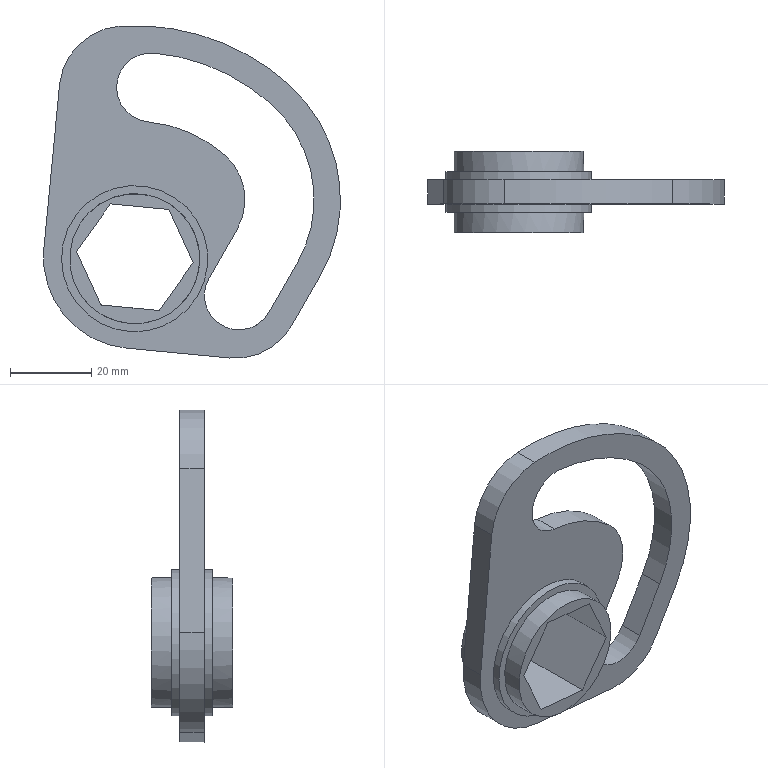Component | NX | ZHUANZHOUTAO | 1 solid | 32 faces | volume 21845 mm3 | plane 17 | cylinder 15 | commonest cylinder face diameters 32 x4 17 x2 36 x2 67 x1 29.077 x1 63.077 x1 101 x1 45 x1